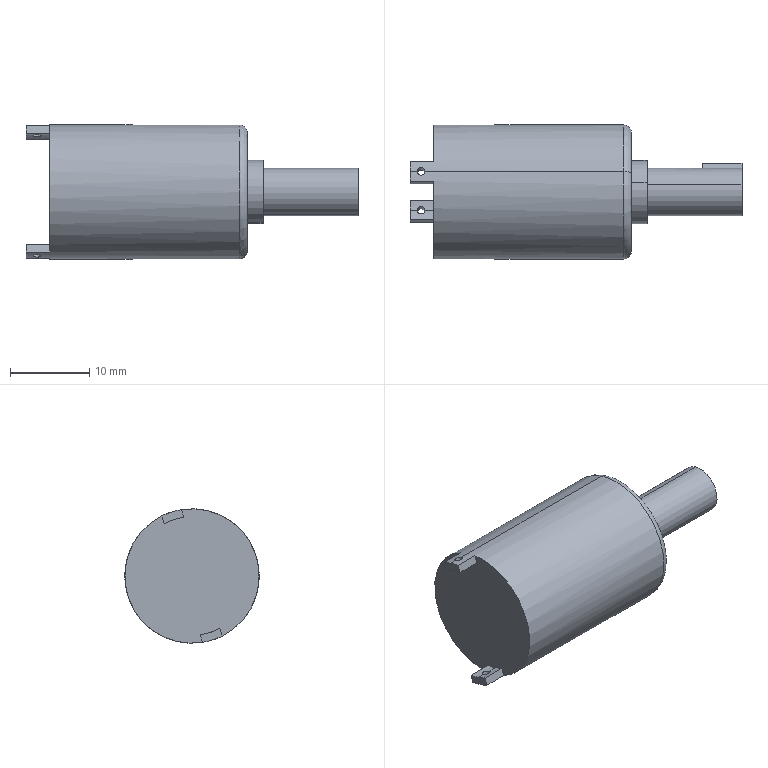Component | SolidWorks | dj-1 | 1 solid | 29 faces | box 42 x 17 x 17 mm | volume 6122 mm3 | plane 14 | cylinder 13 | torus 2 | commonest cylinder face diameters 1 x4 15 x3 6 x2 8 x2 17 x2
build123d program:
from build123d import *
from build123d.topology import SkipClean

# Parameters (mm, degrees)
SKETCH1_R           = 8.5
BOSS_EXTRUDE1_DEPTH = 25
SKETCH2_R           = 4
BOSS_EXTRUDE2_DEPTH = 2
SKETCH3_R           = 3
BOSS_EXTRUDE3_DEPTH = 12
BOSS_EXTRUDE4_START = 3
BOSS_EXTRUDE4_DEPTH = 3
SKETCH5_R           = 0.5
CUT_EXTRUDE1_DEPTH  = 31.5
FILLET1_R           = 1
SKETCH6_W           = 1.566
SKETCH6_H           = 3.572
BOSS_EXTRUDE5_DEPTH = 5


with BuildPart() as part:
    # Sketch1 → Boss-Extrude1 (new body)
    with BuildSketch(Plane.XY):
        Circle(SKETCH1_R)
    extrude(amount=BOSS_EXTRUDE1_DEPTH)

    # Sketch2 → Boss-Extrude2 (add)
    with BuildSketch(Plane.XY.offset(25)):
        Circle(SKETCH2_R)
    extrude(amount=BOSS_EXTRUDE2_DEPTH)

    # Sketch3 → Boss-Extrude3 (add)
    with BuildSketch(Plane.XY.offset(27)):
        with Locations(Location((0, 0, 0), (0, 0, 180))):
            Circle(SKETCH3_R)
    extrude(amount=BOSS_EXTRUDE3_DEPTH)

    # Sketch4 → Boss-Extrude4 (add)
    with SkipClean():  # the faces are left unmerged after this step: merging them gives an invalid solid
        with BuildSketch(Plane(origin=(0, 0, 0), x_dir=(-1, 0, 0), z_dir=(0, 0, -1)).offset(BOSS_EXTRUDE4_START)):
            with BuildLine():
                Line((-7.386, 1.303), (-8.399, 1.303))
                ThreePointArc((-8.399, 1.303), (-8.5, 0), (-8.399, -1.303))
                Line((-8.399, -1.303), (-7.386, -1.303))
                ThreePointArc((-7.386, -1.303), (-7.5, 0), (-7.386, 1.303))
            make_face()
            with BuildLine():
                Line((8.399, 1.303), (7.386, 1.303))
                ThreePointArc((7.386, 1.303), (7.5, 0), (7.386, -1.303))
                Line((7.386, -1.303), (8.399, -1.303))
                ThreePointArc((8.399, -1.303), (8.5, 0), (8.399, 1.303))
            make_face()
        extrude(amount=-BOSS_EXTRUDE4_DEPTH)

    # Sketch5 → Cut-Extrude1 (cut, symmetric)
    with SkipClean():  # the faces are left unmerged after this step: merging them gives an invalid solid
        with BuildSketch(Plane(origin=(0, 0, 0), x_dir=(0, 0, -1), z_dir=(1, 0, 0))):
            with Locations((1.599, 0)):
                Circle(SKETCH5_R)
        extrude(amount=CUT_EXTRUDE1_DEPTH, both=True, mode=Mode.SUBTRACT)

    # Fillet1
    fillet1_edges = [part.edges().sort_by_distance(p)[0] for p in [
        (-8.5, 0, 25),
    ]]
    fillet(fillet1_edges, radius=FILLET1_R)

    # Sketch6 → Boss-Extrude5 (add)
    with SkipClean():  # the faces are left unmerged after this step: merging them gives an invalid solid
        with BuildSketch(Plane.XY.offset(39)):
            with Locations((0, 1.786)):
                Rectangle(SKETCH6_W, SKETCH6_H)
        extrude(amount=-BOSS_EXTRUDE5_DEPTH)


solid = part.part

# Placed as in the assembly
solid = solid.moved(Location((24.669, 8.534, 0), (-17.868, 90, 0)))
STEP:
#1=COLOUR_RGB('',0.7922,0.8196,0.9333);
#2=FILL_AREA_STYLE_COLOUR('',#1);
#3=FILL_AREA_STYLE('',(#2));
#4=SURFACE_STYLE_FILL_AREA(#3);
#5=SURFACE_SIDE_STYLE('',(#4));
#6=SURFACE_STYLE_USAGE(.BOTH.,#5);
#7=PRESENTATION_STYLE_ASSIGNMENT((#6));
#8=CARTESIAN_POINT('',(1.916,0.4387,0.3185));
#9=VERTEX_POINT('',#8);
#10=CARTESIAN_POINT('',(1.916,0.2333,-0.3185));
#11=VERTEX_POINT('',#10);
#12=CARTESIAN_POINT('',(1.916,0.336,-0.));
#13=DIRECTION('',(-1.,0.,0.));
#14=DIRECTION('',(0.,-0.3068,-0.9518));
#15=AXIS2_PLACEMENT_3D('',#12,#13,#14);
#16=CIRCLE('',#15,0.3346);
#17=EDGE_CURVE('',#9,#11,#16,.T.);
#18=ORIENTED_EDGE('',*,*,#17,.F.);
#19=CARTESIAN_POINT('',(1.955,0.4266,0.281));
#20=VERTEX_POINT('',#19);
#21=CARTESIAN_POINT('',(1.916,0.4266,0.281));
#22=DIRECTION('',(0.,0.9518,-0.3068));
#23=DIRECTION('',(0.,0.3068,0.9518));
#24=AXIS2_PLACEMENT_3D('',#21,#22,#23);
#25=CIRCLE('',#24,0.03937);
#26=EDGE_CURVE('',#9,#20,#25,.T.);
#27=ORIENTED_EDGE('',*,*,#26,.T.);
#28=CARTESIAN_POINT('',(1.955,0.2454,-0.281));
#29=VERTEX_POINT('',#28);
#30=CARTESIAN_POINT('',(1.955,0.336,-0.));
#31=DIRECTION('',(1.,0.,0.));
#32=DIRECTION('',(0.,-0.3068,-0.9518));
#33=AXIS2_PLACEMENT_3D('',#30,#31,#32);
#34=CIRCLE('',#33,0.2953);
#35=EDGE_CURVE('',#29,#20,#34,.T.);
#36=ORIENTED_EDGE('',*,*,#35,.F.);
#37=CARTESIAN_POINT('',(1.916,0.2454,-0.281));
#38=DIRECTION('',(0.,-0.9518,0.3068));
#39=DIRECTION('',(0.,-0.3068,-0.9518));
#40=AXIS2_PLACEMENT_3D('',#37,#38,#39);
#41=CIRCLE('',#40,0.03937);
#42=EDGE_CURVE('',#11,#29,#41,.T.);
#43=ORIENTED_EDGE('',*,*,#42,.F.);
#44=EDGE_LOOP('',(#18,#27,#36,#43));
#45=FACE_OUTER_BOUND('',#44,.T.);
#46=CARTESIAN_POINT('',(1.916,0.336,-0.));
#47=DIRECTION('',(1.,0.,0.));
#48=DIRECTION('',(0.,-0.3068,-0.9518));
#49=AXIS2_PLACEMENT_3D('',#46,#47,#48);
#50=TOROIDAL_SURFACE('',#49,0.2953,0.03937);
#51=ADVANCED_FACE('',(#45),#50,.T.);
#52=CARTESIAN_POINT('',(0.928,0.4387,0.3185));
#53=VERTEX_POINT('',#52);
#54=CARTESIAN_POINT('',(0.8886,0.4387,0.3185));
#55=VERTEX_POINT('',#54);
#56=CARTESIAN_POINT('',(0.928,0.4387,0.3185));
#57=CARTESIAN_POINT('',(0.928,0.4337,0.3201));
#58=CARTESIAN_POINT('',(0.9258,0.4288,0.3215));
#59=CARTESIAN_POINT('',(0.9186,0.4218,0.3235));
#60=CARTESIAN_POINT('',(0.9134,0.4197,0.324));
#61=CARTESIAN_POINT('',(0.9031,0.4197,0.324));
#62=CARTESIAN_POINT('',(0.898,0.4218,0.3235));
#63=CARTESIAN_POINT('',(0.8907,0.4289,0.3215));
#64=CARTESIAN_POINT('',(0.8886,0.4338,0.3201));
#65=CARTESIAN_POINT('',(0.8886,0.4387,0.3185));
#66=B_SPLINE_CURVE_WITH_KNOTS('',3,(#56,#57,#58,#59,#60,#61,#62,#63,#64,#65),.UNSPECIFIED.,.F.,.F.,(4,2,2,2,4),(0.,0.0003909,0.0007818,0.001173,0.001564),.UNSPECIFIED.);
#67=EDGE_CURVE('',#53,#55,#66,.T.);
#68=ORIENTED_EDGE('',*,*,#67,.F.);
#69=CARTESIAN_POINT('',(0.928,0.4266,0.281));
#70=VERTEX_POINT('',#69);
#71=CARTESIAN_POINT('',(0.928,0.7165,1.18));
#72=DIRECTION('',(0.,-0.3068,-0.9518));
#73=VECTOR('',#72,39.37);
#74=LINE('',#71,#73);
#75=EDGE_CURVE('',#53,#70,#74,.T.);
#76=ORIENTED_EDGE('',*,*,#75,.T.);
#77=CARTESIAN_POINT('',(0.8886,0.4266,0.281));
#78=VERTEX_POINT('',#77);
#79=CARTESIAN_POINT('',(0.8886,0.4266,0.281));
#80=CARTESIAN_POINT('',(0.8886,0.4216,0.2826));
#81=CARTESIAN_POINT('',(0.8907,0.4167,0.284));
#82=CARTESIAN_POINT('',(0.898,0.4097,0.2859));
#83=CARTESIAN_POINT('',(0.9031,0.4076,0.2864));
#84=CARTESIAN_POINT('',(0.9134,0.4076,0.2864));
#85=CARTESIAN_POINT('',(0.9185,0.4097,0.286));
#86=CARTESIAN_POINT('',(0.9259,0.4168,0.284));
#87=CARTESIAN_POINT('',(0.928,0.4217,0.2826));
#88=CARTESIAN_POINT('',(0.928,0.4266,0.281));
#89=B_SPLINE_CURVE_WITH_KNOTS('',3,(#79,#80,#81,#82,#83,#84,#85,#86,#87,#88),.UNSPECIFIED.,.F.,.F.,(4,2,2,2,4),(0.,0.0003909,0.0007818,0.001173,0.001564),.UNSPECIFIED.);
#90=EDGE_CURVE('',#78,#70,#89,.T.);
#91=ORIENTED_EDGE('',*,*,#90,.F.);
#92=CARTESIAN_POINT('',(0.8886,0.7165,1.18));
#93=DIRECTION('',(0.,-0.3068,-0.9518));
#94=VECTOR('',#93,39.37);
#95=LINE('',#92,#94);
#96=EDGE_CURVE('',#55,#78,#95,.T.);
#97=ORIENTED_EDGE('',*,*,#96,.F.);
#98=EDGE_LOOP('',(#68,#76,#91,#97));
#99=FACE_OUTER_BOUND('',#98,.T.);
#100=CARTESIAN_POINT('',(0.9083,0.7165,1.18));
#101=DIRECTION('',(0.,-0.3068,-0.9518));
#102=DIRECTION('',(-1.,0.,0.));
#103=AXIS2_PLACEMENT_3D('',#100,#101,#102);
#104=CYLINDRICAL_SURFACE('',#103,0.01969);
#105=ADVANCED_FACE('',(#99),#104,.F.);
#106=CARTESIAN_POINT('',(0.928,0.2454,-0.281));
#107=VERTEX_POINT('',#106);
#108=CARTESIAN_POINT('',(0.8886,0.2454,-0.281));
#109=VERTEX_POINT('',#108);
#110=CARTESIAN_POINT('',(0.928,0.2454,-0.281));
#111=CARTESIAN_POINT('',(0.928,0.2405,-0.2795));
#112=CARTESIAN_POINT('',(0.9258,0.2357,-0.2777));
#113=CARTESIAN_POINT('',(0.9186,0.2288,-0.2752));
#114=CARTESIAN_POINT('',(0.9135,0.2269,-0.2744));
#115=CARTESIAN_POINT('',(0.9031,0.2268,-0.2744));
#116=CARTESIAN_POINT('',(0.898,0.2288,-0.2752));
#117=CARTESIAN_POINT('',(0.8907,0.2356,-0.2777));
#118=CARTESIAN_POINT('',(0.8886,0.2404,-0.2794));
#119=CARTESIAN_POINT('',(0.8886,0.2454,-0.281));
#120=B_SPLINE_CURVE_WITH_KNOTS('',3,(#110,#111,#112,#113,#114,#115,#116,#117,#118,#119),.UNSPECIFIED.,.F.,.F.,(4,2,2,2,4),(0.001564,0.001954,0.002345,0.002736,0.003127),.UNSPECIFIED.);
#121=EDGE_CURVE('',#107,#109,#120,.T.);
#122=ORIENTED_EDGE('',*,*,#121,.F.);
#123=CARTESIAN_POINT('',(0.928,0.2333,-0.3185));
#124=VERTEX_POINT('',#123);
#125=CARTESIAN_POINT('',(0.928,0.7165,1.18));
#126=DIRECTION('',(0.,-0.3068,-0.9518));
#127=VECTOR('',#126,39.37);
#128=LINE('',#125,#127);
#129=EDGE_CURVE('',#107,#124,#128,.T.);
#130=ORIENTED_EDGE('',*,*,#129,.T.);
#131=CARTESIAN_POINT('',(0.8886,0.2333,-0.3185));
#132=VERTEX_POINT('',#131);
#133=CARTESIAN_POINT('',(0.8886,0.2333,-0.3185));
#134=CARTESIAN_POINT('',(0.8886,0.2284,-0.3169));
#135=CARTESIAN_POINT('',(0.8907,0.2236,-0.3152));
#136=CARTESIAN_POINT('',(0.898,0.2167,-0.3127));
#137=CARTESIAN_POINT('',(0.9031,0.2147,-0.3119));
#138=CARTESIAN_POINT('',(0.9134,0.2147,-0.3119));
#139=CARTESIAN_POINT('',(0.9185,0.2167,-0.3127));
#140=CARTESIAN_POINT('',(0.9259,0.2236,-0.3152));
#141=CARTESIAN_POINT('',(0.928,0.2284,-0.3169));
#142=CARTESIAN_POINT('',(0.928,0.2333,-0.3185));
#143=B_SPLINE_CURVE_WITH_KNOTS('',3,(#133,#134,#135,#136,#137,#138,#139,#140,#141,#142),.UNSPECIFIED.,.F.,.F.,(4,2,2,2,4),(0.,0.0003909,0.0007818,0.001173,0.001564),.UNSPECIFIED.);
#144=EDGE_CURVE('',#132,#124,#143,.T.);
#145=ORIENTED_EDGE('',*,*,#144,.F.);
#146=CARTESIAN_POINT('',(0.8886,0.7165,1.18));
#147=DIRECTION('',(0.,-0.3068,-0.9518));
#148=VECTOR('',#147,39.37);
#149=LINE('',#146,#148);
#150=EDGE_CURVE('',#109,#132,#149,.T.);
#151=ORIENTED_EDGE('',*,*,#150,.F.);
#152=EDGE_LOOP('',(#122,#130,#145,#151));
#153=FACE_OUTER_BOUND('',#152,.T.);
#154=CARTESIAN_POINT('',(0.9083,0.7165,1.18));
#155=DIRECTION('',(0.,-0.3068,-0.9518));
#156=DIRECTION('',(-1.,0.,0.));
#157=AXIS2_PLACEMENT_3D('',#154,#155,#156);
#158=CYLINDRICAL_SURFACE('',#157,0.01969);
#159=ADVANCED_FACE('',(#153),#158,.F.);
#160=CARTESIAN_POINT('',(0.8531,0.2454,-0.281));
#161=VERTEX_POINT('',#160);
#162=CARTESIAN_POINT('',(0.8531,0.2956,-0.2925));
#163=VERTEX_POINT('',#162);
#164=CARTESIAN_POINT('',(0.8531,0.336,-0.));
#165=DIRECTION('',(1.,0.,0.));
#166=DIRECTION('',(0.,0.3068,0.9518));
#167=AXIS2_PLACEMENT_3D('',#164,#165,#166);
#168=CIRCLE('',#167,0.2953);
#169=EDGE_CURVE('',#161,#163,#168,.T.);
#170=ORIENTED_EDGE('',*,*,#169,.F.);
#171=CARTESIAN_POINT('',(0.8531,0.2454,-0.281));
#172=DIRECTION('',(1.,0.,0.));
#173=VECTOR('',#172,39.37);
#174=LINE('',#171,#173);
#175=EDGE_CURVE('',#161,#109,#174,.T.);
#176=ORIENTED_EDGE('',*,*,#175,.T.);
#177=CARTESIAN_POINT('',(0.8886,0.2454,-0.281));
#178=CARTESIAN_POINT('',(0.8886,0.2503,-0.2826));
#179=CARTESIAN_POINT('',(0.8907,0.2552,-0.284));
#180=CARTESIAN_POINT('',(0.898,0.2622,-0.2859));
#181=CARTESIAN_POINT('',(0.9031,0.2643,-0.2864));
#182=CARTESIAN_POINT('',(0.9134,0.2643,-0.2864));
#183=CARTESIAN_POINT('',(0.9185,0.2623,-0.286));
#184=CARTESIAN_POINT('',(0.9259,0.2552,-0.284));
#185=CARTESIAN_POINT('',(0.928,0.2503,-0.2826));
#186=CARTESIAN_POINT('',(0.928,0.2454,-0.281));
#187=B_SPLINE_CURVE_WITH_KNOTS('',3,(#177,#178,#179,#180,#181,#182,#183,#184,#185,#186),.UNSPECIFIED.,.F.,.F.,(4,2,2,2,4),(0.,0.0003909,0.0007818,0.001173,0.001564),.UNSPECIFIED.);
#188=EDGE_CURVE('',#109,#107,#187,.T.);
#189=ORIENTED_EDGE('',*,*,#188,.T.);
#190=CARTESIAN_POINT('',(0.9712,0.2454,-0.281));
#191=VERTEX_POINT('',#190);
#192=CARTESIAN_POINT('',(0.8531,0.2454,-0.281));
#193=DIRECTION('',(1.,0.,0.));
#194=VECTOR('',#193,39.37);
#195=LINE('',#192,#194);
#196=EDGE_CURVE('',#107,#191,#195,.T.);
#197=ORIENTED_EDGE('',*,*,#196,.T.);
#198=CARTESIAN_POINT('',(0.9712,0.2956,-0.2925));
#199=VERTEX_POINT('',#198);
#200=CARTESIAN_POINT('',(0.9712,0.336,-0.));
#201=DIRECTION('',(1.,0.,0.));
#202=DIRECTION('',(0.,0.3068,0.9518));
#203=AXIS2_PLACEMENT_3D('',#200,#201,#202);
#204=CIRCLE('',#203,0.2953);
#205=EDGE_CURVE('',#191,#199,#204,.T.);
#206=ORIENTED_EDGE('',*,*,#205,.T.);
#207=CARTESIAN_POINT('',(0.8531,0.2956,-0.2925));
#208=DIRECTION('',(1.,0.,0.));
#209=VECTOR('',#208,39.37);
#210=LINE('',#207,#209);
#211=EDGE_CURVE('',#163,#199,#210,.T.);
#212=ORIENTED_EDGE('',*,*,#211,.F.);
#213=EDGE_LOOP('',(#170,#176,#189,#197,#206,#212));
#214=FACE_OUTER_BOUND('',#213,.T.);
#215=CARTESIAN_POINT('',(0.8531,0.336,-0.));
#216=DIRECTION('',(1.,0.,0.));
#217=DIRECTION('',(0.,-0.3068,-0.9518));
#218=AXIS2_PLACEMENT_3D('',#215,#216,#217);
#219=CYLINDRICAL_SURFACE('',#218,0.2953);
#220=ADVANCED_FACE('',(#214),#219,.F.);
#221=CARTESIAN_POINT('',(2.507,0.2997,-0.1124));
#222=VERTEX_POINT('',#221);
#223=CARTESIAN_POINT('',(2.507,0.435,-0.06432));
#224=VERTEX_POINT('',#223);
#225=CARTESIAN_POINT('',(2.507,0.336,-0.));
#226=DIRECTION('',(1.,0.,0.));
#227=DIRECTION('',(0.,-0.3068,-0.9518));
#228=AXIS2_PLACEMENT_3D('',#225,#226,#227);
#229=CIRCLE('',#228,0.1181);
#230=EDGE_CURVE('',#222,#224,#229,.T.);
#231=ORIENTED_EDGE('',*,*,#230,.F.);
#232=CARTESIAN_POINT('',(2.034,0.2997,-0.1124));
#233=VERTEX_POINT('',#232);
#234=CARTESIAN_POINT('',(2.507,0.2997,-0.1124));
#235=DIRECTION('',(-1.,0.,0.));
#236=VECTOR('',#235,39.37);
#237=LINE('',#234,#236);
#238=EDGE_CURVE('',#222,#233,#237,.T.);
#239=ORIENTED_EDGE('',*,*,#238,.T.);
#240=CARTESIAN_POINT('',(2.034,0.3722,0.1124));
#241=VERTEX_POINT('',#240);
#242=CARTESIAN_POINT('',(2.034,0.336,-0.));
#243=DIRECTION('',(1.,0.,0.));
#244=DIRECTION('',(0.,-0.3068,-0.9518));
#245=AXIS2_PLACEMENT_3D('',#242,#243,#244);
#246=CIRCLE('',#245,0.1181);
#247=EDGE_CURVE('',#233,#241,#246,.T.);
#248=ORIENTED_EDGE('',*,*,#247,.T.);
#249=CARTESIAN_POINT('',(2.507,0.3722,0.1124));
#250=VERTEX_POINT('',#249);
#251=CARTESIAN_POINT('',(2.507,0.3722,0.1124));
#252=DIRECTION('',(-1.,0.,0.));
#253=VECTOR('',#252,39.37);
#254=LINE('',#251,#253);
#255=EDGE_CURVE('',#250,#241,#254,.T.);
#256=ORIENTED_EDGE('',*,*,#255,.F.);
#257=CARTESIAN_POINT('',(2.507,0.454,-0.005646));
#258=VERTEX_POINT('',#257);
#259=CARTESIAN_POINT('',(2.507,0.336,-0.));
#260=DIRECTION('',(1.,0.,0.));
#261=DIRECTION('',(0.,-0.3068,-0.9518));
#262=AXIS2_PLACEMENT_3D('',#259,#260,#261);
#263=CIRCLE('',#262,0.1181);
#264=EDGE_CURVE('',#258,#250,#263,.T.);
#265=ORIENTED_EDGE('',*,*,#264,.F.);
#266=CARTESIAN_POINT('',(2.31,0.454,-0.005646));
#267=VERTEX_POINT('',#266);
#268=CARTESIAN_POINT('',(2.507,0.454,-0.005646));
#269=DIRECTION('',(-1.,0.,0.));
#270=VECTOR('',#269,39.37);
#271=LINE('',#268,#270);
#272=EDGE_CURVE('',#258,#267,#271,.T.);
#273=ORIENTED_EDGE('',*,*,#272,.T.);
#274=CARTESIAN_POINT('',(2.31,0.435,-0.06432));
#275=VERTEX_POINT('',#274);
#276=CARTESIAN_POINT('',(2.31,0.336,-0.));
#277=DIRECTION('',(1.,0.,0.));
#278=DIRECTION('',(0.,-0.3068,-0.9518));
#279=AXIS2_PLACEMENT_3D('',#276,#277,#278);
#280=CIRCLE('',#279,0.1181);
#281=EDGE_CURVE('',#275,#267,#280,.T.);
#282=ORIENTED_EDGE('',*,*,#281,.F.);
#283=CARTESIAN_POINT('',(2.507,0.435,-0.06432));
#284=DIRECTION('',(1.,0.,0.));
#285=VECTOR('',#284,39.37);
#286=LINE('',#283,#285);
#287=EDGE_CURVE('',#275,#224,#286,.T.);
#288=ORIENTED_EDGE('',*,*,#287,.T.);
#289=EDGE_LOOP('',(#231,#239,#248,#256,#265,#273,#282,#288));
#290=FACE_OUTER_BOUND('',#289,.T.);
#291=CARTESIAN_POINT('',(2.507,0.336,-0.));
#292=DIRECTION('',(-1.,0.,0.));
#293=DIRECTION('',(0.,0.3068,0.9518));
#294=AXIS2_PLACEMENT_3D('',#291,#292,#293);
#295=CYLINDRICAL_SURFACE('',#294,0.1181);
#296=ADVANCED_FACE('',(#290),#295,.T.);
#297=CARTESIAN_POINT('',(2.034,0.2877,-0.1499));
#298=VERTEX_POINT('',#297);
#299=CARTESIAN_POINT('',(2.034,0.3843,0.1499));
#300=VERTEX_POINT('',#299);
#301=CARTESIAN_POINT('',(2.034,0.336,-0.));
#302=DIRECTION('',(1.,0.,0.));
#303=DIRECTION('',(0.,-0.3068,-0.9518));
#304=AXIS2_PLACEMENT_3D('',#301,#302,#303);
#305=CIRCLE('',#304,0.1575);
#306=EDGE_CURVE('',#298,#300,#305,.T.);
#307=ORIENTED_EDGE('',*,*,#306,.F.);
#308=CARTESIAN_POINT('',(1.955,0.2877,-0.1499));
#309=VERTEX_POINT('',#308);
#310=CARTESIAN_POINT('',(2.034,0.2877,-0.1499));
#311=DIRECTION('',(-1.,0.,0.));
#312=VECTOR('',#311,39.37);
#313=LINE('',#310,#312);
#314=EDGE_CURVE('',#298,#309,#313,.T.);
#315=ORIENTED_EDGE('',*,*,#314,.T.);
#316=CARTESIAN_POINT('',(1.955,0.3843,0.1499));
#317=VERTEX_POINT('',#316);
#318=CARTESIAN_POINT('',(1.955,0.336,-0.));
#319=DIRECTION('',(1.,0.,0.));
#320=DIRECTION('',(0.,-0.3068,-0.9518));
#321=AXIS2_PLACEMENT_3D('',#318,#319,#320);
#322=CIRCLE('',#321,0.1575);
#323=EDGE_CURVE('',#309,#317,#322,.T.);
#324=ORIENTED_EDGE('',*,*,#323,.T.);
#325=CARTESIAN_POINT('',(2.034,0.3843,0.1499));
#326=DIRECTION('',(-1.,0.,0.));
#327=VECTOR('',#326,39.37);
#328=LINE('',#325,#327);
#329=EDGE_CURVE('',#300,#317,#328,.T.);
#330=ORIENTED_EDGE('',*,*,#329,.F.);
#331=EDGE_LOOP('',(#307,#315,#324,#330));
#332=FACE_OUTER_BOUND('',#331,.T.);
#333=CARTESIAN_POINT('',(2.034,0.336,-0.));
#334=DIRECTION('',(-1.,0.,0.));
#335=DIRECTION('',(0.,0.3068,0.9518));
#336=AXIS2_PLACEMENT_3D('',#333,#334,#335);
#337=CYLINDRICAL_SURFACE('',#336,0.1575);
#338=ADVANCED_FACE('',(#332),#337,.T.);
#339=ORIENTED_EDGE('',*,*,#17,.T.);
#340=CARTESIAN_POINT('',(1.955,0.2333,-0.3185));
#341=DIRECTION('',(-1.,0.,0.));
#342=VECTOR('',#341,39.37);
#343=LINE('',#340,#342);
#344=EDGE_CURVE('',#11,#124,#343,.T.);
#345=ORIENTED_EDGE('',*,*,#344,.T.);
#346=CARTESIAN_POINT('',(0.928,0.2333,-0.3185));
#347=CARTESIAN_POINT('',(0.928,0.2382,-0.3201));
#348=CARTESIAN_POINT('',(0.9258,0.2431,-0.3215));
#349=CARTESIAN_POINT('',(0.9186,0.2501,-0.3235));
#350=CARTESIAN_POINT('',(0.9135,0.2522,-0.324));
#351=CARTESIAN_POINT('',(0.9031,0.2522,-0.324));
#352=CARTESIAN_POINT('',(0.898,0.2502,-0.3235));
#353=CARTESIAN_POINT('',(0.8907,0.2431,-0.3215));
#354=CARTESIAN_POINT('',(0.8886,0.2383,-0.3201));
#355=CARTESIAN_POINT('',(0.8886,0.2333,-0.3185));
#356=B_SPLINE_CURVE_WITH_KNOTS('',3,(#346,#347,#348,#349,#350,#351,#352,#353,#354,#355),.UNSPECIFIED.,.F.,.F.,(4,2,2,2,4),(0.001564,0.001954,0.002345,0.002736,0.003127),.UNSPECIFIED.);
#357=EDGE_CURVE('',#124,#132,#356,.T.);
#358=ORIENTED_EDGE('',*,*,#357,.T.);
#359=CARTESIAN_POINT('',(0.8531,0.2333,-0.3185));
#360=VERTEX_POINT('',#359);
#361=CARTESIAN_POINT('',(1.955,0.2333,-0.3185));
#362=DIRECTION('',(-1.,0.,0.));
#363=VECTOR('',#362,39.37);
#364=LINE('',#361,#363);
#365=EDGE_CURVE('',#132,#360,#364,.T.);
#366=ORIENTED_EDGE('',*,*,#365,.T.);
#367=CARTESIAN_POINT('',(0.8531,0.2834,-0.3305));
#368=VERTEX_POINT('',#367);
#369=CARTESIAN_POINT('',(0.8531,0.336,-0.));
#370=DIRECTION('',(-1.,0.,0.));
#371=DIRECTION('',(0.,0.3068,0.9518));
#372=AXIS2_PLACEMENT_3D('',#369,#370,#371);
#373=CIRCLE('',#372,0.3346);
#374=EDGE_CURVE('',#368,#360,#373,.T.);
#375=ORIENTED_EDGE('',*,*,#374,.F.);
#376=CARTESIAN_POINT('',(0.9712,0.2834,-0.3305));
#377=VERTEX_POINT('',#376);
#378=CARTESIAN_POINT('',(0.8531,0.2834,-0.3305));
#379=DIRECTION('',(1.,0.,0.));
#380=VECTOR('',#379,39.37);
#381=LINE('',#378,#380);
#382=EDGE_CURVE('',#368,#377,#381,.T.);
#383=ORIENTED_EDGE('',*,*,#382,.T.);
#384=CARTESIAN_POINT('',(0.9712,0.4863,0.299));
#385=VERTEX_POINT('',#384);
#386=CARTESIAN_POINT('',(0.9712,0.336,-0.));
#387=DIRECTION('',(1.,0.,0.));
#388=DIRECTION('',(0.,-0.3068,-0.9518));
#389=AXIS2_PLACEMENT_3D('',#386,#387,#388);
#390=CIRCLE('',#389,0.3346);
#391=EDGE_CURVE('',#377,#385,#390,.T.);
#392=ORIENTED_EDGE('',*,*,#391,.T.);
#393=CARTESIAN_POINT('',(0.8531,0.4863,0.299));
#394=VERTEX_POINT('',#393);
#395=CARTESIAN_POINT('',(0.8531,0.4863,0.299));
#396=DIRECTION('',(1.,0.,0.));
#397=VECTOR('',#396,39.37);
#398=LINE('',#395,#397);
#399=EDGE_CURVE('',#394,#385,#398,.T.);
#400=ORIENTED_EDGE('',*,*,#399,.F.);
#401=CARTESIAN_POINT('',(0.8531,0.4387,0.3185));
#402=VERTEX_POINT('',#401);
#403=CARTESIAN_POINT('',(0.8531,0.336,-0.));
#404=DIRECTION('',(-1.,0.,0.));
#405=DIRECTION('',(0.,0.3068,0.9518));
#406=AXIS2_PLACEMENT_3D('',#403,#404,#405);
#407=CIRCLE('',#406,0.3346);
#408=EDGE_CURVE('',#402,#394,#407,.T.);
#409=ORIENTED_EDGE('',*,*,#408,.F.);
#410=CARTESIAN_POINT('',(1.955,0.4387,0.3185));
#411=DIRECTION('',(-1.,0.,0.));
#412=VECTOR('',#411,39.37);
#413=LINE('',#410,#412);
#414=EDGE_CURVE('',#55,#402,#413,.T.);
#415=ORIENTED_EDGE('',*,*,#414,.F.);
#416=CARTESIAN_POINT('',(0.8886,0.4387,0.3185));
#417=CARTESIAN_POINT('',(0.8886,0.4436,0.3169));
#418=CARTESIAN_POINT('',(0.8907,0.4484,0.3152));
#419=CARTESIAN_POINT('',(0.898,0.4552,0.3127));
#420=CARTESIAN_POINT('',(0.9031,0.4572,0.3119));
#421=CARTESIAN_POINT('',(0.9135,0.4572,0.3119));
#422=CARTESIAN_POINT('',(0.9185,0.4552,0.3127));
#423=CARTESIAN_POINT('',(0.9258,0.4484,0.3152));
#424=CARTESIAN_POINT('',(0.928,0.4436,0.3169));
#425=CARTESIAN_POINT('',(0.928,0.4387,0.3185));
#426=B_SPLINE_CURVE_WITH_KNOTS('',3,(#416,#417,#418,#419,#420,#421,#422,#423,#424,#425),.UNSPECIFIED.,.F.,.F.,(4,2,2,2,4),(0.001564,0.001954,0.002345,0.002736,0.003127),.UNSPECIFIED.);
#427=EDGE_CURVE('',#55,#53,#426,.T.);
#428=ORIENTED_EDGE('',*,*,#427,.T.);
#429=CARTESIAN_POINT('',(1.955,0.4387,0.3185));
#430=DIRECTION('',(-1.,0.,0.));
#431=VECTOR('',#430,39.37);
#432=LINE('',#429,#431);
#433=EDGE_CURVE('',#9,#53,#432,.T.);
#434=ORIENTED_EDGE('',*,*,#433,.F.);
#435=EDGE_LOOP('',(#339,#345,#358,#366,#375,#383,#392,#400,#409,#415,#428,#434));
#436=FACE_OUTER_BOUND('',#435,.T.);
#437=CARTESIAN_POINT('',(1.955,0.336,-0.));
#438=DIRECTION('',(-1.,0.,0.));
#439=DIRECTION('',(0.,0.3068,0.9518));
#440=AXIS2_PLACEMENT_3D('',#437,#438,#439);
#441=CYLINDRICAL_SURFACE('',#440,0.3346);
#442=ADVANCED_FACE('',(#436),#441,.T.);
#443=CARTESIAN_POINT('',(0.9712,0.1857,-0.299));
#444=VERTEX_POINT('',#443);
#445=CARTESIAN_POINT('',(0.9712,0.1979,-0.261));
#446=VERTEX_POINT('',#445);
#447=CARTESIAN_POINT('',(0.9712,0.1979,-0.261));
#448=DIRECTION('',(0.,0.3068,0.9518));
#449=VECTOR('',#448,39.37);
#450=LINE('',#447,#449);
#451=EDGE_CURVE('',#444,#446,#450,.T.);
#452=ORIENTED_EDGE('',*,*,#451,.F.);
#453=CARTESIAN_POINT('',(0.9712,0.3886,0.3305));
#454=VERTEX_POINT('',#453);
#455=CARTESIAN_POINT('',(0.9712,0.336,-0.));
#456=DIRECTION('',(1.,0.,0.));
#457=DIRECTION('',(0.,-0.3068,-0.9518));
#458=AXIS2_PLACEMENT_3D('',#455,#456,#457);
#459=CIRCLE('',#458,0.3346);
#460=EDGE_CURVE('',#454,#444,#459,.T.);
#461=ORIENTED_EDGE('',*,*,#460,.F.);
#462=CARTESIAN_POINT('',(0.9712,0.3764,0.2925));
#463=VERTEX_POINT('',#462);
#464=CARTESIAN_POINT('',(0.9712,0.3886,0.3305));
#465=DIRECTION('',(0.,0.3068,0.9518));
#466=VECTOR('',#465,39.37);
#467=LINE('',#464,#466);
#468=EDGE_CURVE('',#463,#454,#467,.T.);
#469=ORIENTED_EDGE('',*,*,#468,.F.);
#470=CARTESIAN_POINT('',(0.9712,0.474,0.261));
#471=VERTEX_POINT('',#470);
#472=CARTESIAN_POINT('',(0.9712,0.336,-0.));
#473=DIRECTION('',(1.,0.,0.));
#474=DIRECTION('',(0.,0.3068,0.9518));
#475=AXIS2_PLACEMENT_3D('',#472,#473,#474);
#476=CIRCLE('',#475,0.2953);
#477=EDGE_CURVE('',#471,#463,#476,.T.);
#478=ORIENTED_EDGE('',*,*,#477,.F.);
#479=CARTESIAN_POINT('',(0.9712,0.4863,0.299));
#480=DIRECTION('',(0.,-0.3068,-0.9518));
#481=VECTOR('',#480,39.37);
#482=LINE('',#479,#481);
#483=EDGE_CURVE('',#385,#471,#482,.T.);
#484=ORIENTED_EDGE('',*,*,#483,.F.);
#485=ORIENTED_EDGE('',*,*,#391,.F.);
#486=CARTESIAN_POINT('',(0.9712,0.2956,-0.2925));
#487=DIRECTION('',(0.,-0.3068,-0.9518));
#488=VECTOR('',#487,39.37);
#489=LINE('',#486,#488);
#490=EDGE_CURVE('',#199,#377,#489,.T.);
#491=ORIENTED_EDGE('',*,*,#490,.F.);
#492=ORIENTED_EDGE('',*,*,#205,.F.);
#493=CARTESIAN_POINT('',(0.9712,0.336,-0.));
#494=DIRECTION('',(1.,0.,0.));
#495=DIRECTION('',(0.,0.3068,0.9518));
#496=AXIS2_PLACEMENT_3D('',#493,#494,#495);
#497=CIRCLE('',#496,0.2953);
#498=EDGE_CURVE('',#446,#191,#497,.T.);
#499=ORIENTED_EDGE('',*,*,#498,.F.);
#500=EDGE_LOOP('',(#452,#461,#469,#478,#484,#485,#491,#492,#499));
#501=FACE_OUTER_BOUND('',#500,.T.);
#502=CARTESIAN_POINT('',(0.9712,0.336,-0.));
#503=DIRECTION('',(1.,0.,0.));
#504=DIRECTION('',(0.,-0.3068,-0.9518));
#505=AXIS2_PLACEMENT_3D('',#502,#503,#504);
#506=PLANE('',#505);
#507=ADVANCED_FACE('',(#501),#506,.F.);
#508=CARTESIAN_POINT('',(2.034,0.336,-0.));
#509=DIRECTION('',(1.,0.,0.));
#510=DIRECTION('',(0.,-0.3068,-0.9518));
#511=AXIS2_PLACEMENT_3D('',#508,#509,#510);
#512=CIRCLE('',#511,0.1575);
#513=EDGE_CURVE('',#300,#298,#512,.T.);
#514=ORIENTED_EDGE('',*,*,#513,.T.);
#515=ORIENTED_EDGE('',*,*,#306,.T.);
#516=EDGE_LOOP('',(#514,#515));
#517=FACE_OUTER_BOUND('',#516,.T.);
#518=CARTESIAN_POINT('',(2.034,0.336,-0.));
#519=DIRECTION('',(1.,0.,0.));
#520=DIRECTION('',(0.,-0.3068,-0.9518));
#521=AXIS2_PLACEMENT_3D('',#518,#519,#520);
#522=CIRCLE('',#521,0.1181);
#523=EDGE_CURVE('',#241,#233,#522,.T.);
#524=ORIENTED_EDGE('',*,*,#523,.F.);
#525=ORIENTED_EDGE('',*,*,#247,.F.);
#526=EDGE_LOOP('',(#524,#525));
#527=FACE_BOUND('',#526,.T.);
#528=CARTESIAN_POINT('',(2.034,0.336,-0.));
#529=DIRECTION('',(1.,0.,0.));
#530=DIRECTION('',(0.,-0.3068,-0.9518));
#531=AXIS2_PLACEMENT_3D('',#528,#529,#530);
#532=PLANE('',#531);
#533=ADVANCED_FACE('',(#517,#527),#532,.T.);
#534=ORIENTED_EDGE('',*,*,#35,.T.);
#535=CARTESIAN_POINT('',(1.955,0.336,-0.));
#536=DIRECTION('',(1.,0.,0.));
#537=DIRECTION('',(0.,-0.3068,-0.9518));
#538=AXIS2_PLACEMENT_3D('',#535,#536,#537);
#539=CIRCLE('',#538,0.2953);
#540=EDGE_CURVE('',#20,#29,#539,.T.);
#541=ORIENTED_EDGE('',*,*,#540,.T.);
#542=EDGE_LOOP('',(#534,#541));
#543=FACE_OUTER_BOUND('',#542,.T.);
#544=CARTESIAN_POINT('',(1.955,0.336,-0.));
#545=DIRECTION('',(1.,0.,0.));
#546=DIRECTION('',(0.,-0.3068,-0.9518));
#547=AXIS2_PLACEMENT_3D('',#544,#545,#546);
#548=CIRCLE('',#547,0.1575);
#549=EDGE_CURVE('',#317,#309,#548,.T.);
#550=ORIENTED_EDGE('',*,*,#549,.F.);
#551=ORIENTED_EDGE('',*,*,#323,.F.);
#552=EDGE_LOOP('',(#550,#551));
#553=FACE_BOUND('',#552,.T.);
#554=CARTESIAN_POINT('',(1.955,0.336,-0.));
#555=DIRECTION('',(1.,0.,0.));
#556=DIRECTION('',(0.,-0.3068,-0.9518));
#557=AXIS2_PLACEMENT_3D('',#554,#555,#556);
#558=PLANE('',#557);
#559=ADVANCED_FACE('',(#543,#553),#558,.T.);
#560=ORIENTED_EDGE('',*,*,#344,.F.);
#561=CARTESIAN_POINT('',(1.916,0.336,-0.));
#562=DIRECTION('',(-1.,0.,0.));
#563=DIRECTION('',(0.,-0.3068,-0.9518));
#564=AXIS2_PLACEMENT_3D('',#561,#562,#563);
#565=CIRCLE('',#564,0.3346);
#566=EDGE_CURVE('',#11,#9,#565,.T.);
#567=ORIENTED_EDGE('',*,*,#566,.T.);
#568=ORIENTED_EDGE('',*,*,#433,.T.);
#569=ORIENTED_EDGE('',*,*,#67,.T.);
#570=ORIENTED_EDGE('',*,*,#414,.T.);
#571=CARTESIAN_POINT('',(0.8531,0.3886,0.3305));
#572=VERTEX_POINT('',#571);
#573=CARTESIAN_POINT('',(0.8531,0.336,-0.));
#574=DIRECTION('',(-1.,0.,0.));
#575=DIRECTION('',(0.,0.3068,0.9518));
#576=AXIS2_PLACEMENT_3D('',#573,#574,#575);
#577=CIRCLE('',#576,0.3346);
#578=EDGE_CURVE('',#572,#402,#577,.T.);
#579=ORIENTED_EDGE('',*,*,#578,.F.);
#580=CARTESIAN_POINT('',(0.8531,0.3886,0.3305));
#581=DIRECTION('',(1.,0.,0.));
#582=VECTOR('',#581,39.37);
#583=LINE('',#580,#582);
#584=EDGE_CURVE('',#572,#454,#583,.T.);
#585=ORIENTED_EDGE('',*,*,#584,.T.);
#586=ORIENTED_EDGE('',*,*,#460,.T.);
#587=CARTESIAN_POINT('',(0.8531,0.1857,-0.299));
#588=VERTEX_POINT('',#587);
#589=CARTESIAN_POINT('',(0.8531,0.1857,-0.299));
#590=DIRECTION('',(1.,0.,0.));
#591=VECTOR('',#590,39.37);
#592=LINE('',#589,#591);
#593=EDGE_CURVE('',#588,#444,#592,.T.);
#594=ORIENTED_EDGE('',*,*,#593,.F.);
#595=CARTESIAN_POINT('',(0.8531,0.336,-0.));
#596=DIRECTION('',(-1.,0.,0.));
#597=DIRECTION('',(0.,0.3068,0.9518));
#598=AXIS2_PLACEMENT_3D('',#595,#596,#597);
#599=CIRCLE('',#598,0.3346);
#600=EDGE_CURVE('',#360,#588,#599,.T.);
#601=ORIENTED_EDGE('',*,*,#600,.F.);
#602=ORIENTED_EDGE('',*,*,#365,.F.);
#603=ORIENTED_EDGE('',*,*,#144,.T.);
#604=EDGE_LOOP('',(#560,#567,#568,#569,#570,#579,#585,#586,#594,#601,#602,#603));
#605=FACE_OUTER_BOUND('',#604,.T.);
#606=CARTESIAN_POINT('',(1.955,0.336,-0.));
#607=DIRECTION('',(-1.,0.,0.));
#608=DIRECTION('',(0.,0.3068,0.9518));
#609=AXIS2_PLACEMENT_3D('',#606,#607,#608);
#610=CYLINDRICAL_SURFACE('',#609,0.3346);
#611=ADVANCED_FACE('',(#605),#610,.T.);
#612=ORIENTED_EDGE('',*,*,#314,.F.);
#613=ORIENTED_EDGE('',*,*,#513,.F.);
#614=ORIENTED_EDGE('',*,*,#329,.T.);
#615=ORIENTED_EDGE('',*,*,#549,.T.);
#616=EDGE_LOOP('',(#612,#613,#614,#615));
#617=FACE_OUTER_BOUND('',#616,.T.);
#618=CARTESIAN_POINT('',(2.034,0.336,-0.));
#619=DIRECTION('',(-1.,0.,0.));
#620=DIRECTION('',(0.,0.3068,0.9518));
#621=AXIS2_PLACEMENT_3D('',#618,#619,#620);
#622=CYLINDRICAL_SURFACE('',#621,0.1575);
#623=ADVANCED_FACE('',(#617),#622,.T.);
#624=ORIENTED_EDGE('',*,*,#238,.F.);
#625=CARTESIAN_POINT('',(2.507,0.336,-0.));
#626=DIRECTION('',(1.,0.,0.));
#627=DIRECTION('',(0.,-0.3068,-0.9518));
#628=AXIS2_PLACEMENT_3D('',#625,#626,#627);
#629=CIRCLE('',#628,0.1181);
#630=EDGE_CURVE('',#250,#222,#629,.T.);
#631=ORIENTED_EDGE('',*,*,#630,.F.);
#632=ORIENTED_EDGE('',*,*,#255,.T.);
#633=ORIENTED_EDGE('',*,*,#523,.T.);
#634=EDGE_LOOP('',(#624,#631,#632,#633));
#635=FACE_OUTER_BOUND('',#634,.T.);
#636=CARTESIAN_POINT('',(2.507,0.336,-0.));
#637=DIRECTION('',(-1.,0.,0.));
#638=DIRECTION('',(0.,0.3068,0.9518));
#639=AXIS2_PLACEMENT_3D('',#636,#637,#638);
#640=CYLINDRICAL_SURFACE('',#639,0.1181);
#641=ADVANCED_FACE('',(#635),#640,.T.);
#642=ORIENTED_EDGE('',*,*,#264,.T.);
#643=ORIENTED_EDGE('',*,*,#630,.T.);
#644=ORIENTED_EDGE('',*,*,#230,.T.);
#645=CARTESIAN_POINT('',(2.507,0.4604,-0.07249));
#646=VERTEX_POINT('',#645);
#647=CARTESIAN_POINT('',(2.507,0.3265,-0.02934));
#648=DIRECTION('',(0.,0.9518,-0.3068));
#649=VECTOR('',#648,39.37);
#650=LINE('',#647,#649);
#651=EDGE_CURVE('',#224,#646,#650,.T.);
#652=ORIENTED_EDGE('',*,*,#651,.T.);
#653=CARTESIAN_POINT('',(2.507,0.4793,-0.01382));
#654=VERTEX_POINT('',#653);
#655=CARTESIAN_POINT('',(2.507,0.4604,-0.07249));
#656=DIRECTION('',(0.,0.3068,0.9518));
#657=VECTOR('',#656,39.37);
#658=LINE('',#655,#657);
#659=EDGE_CURVE('',#646,#654,#658,.T.);
#660=ORIENTED_EDGE('',*,*,#659,.T.);
#661=CARTESIAN_POINT('',(2.507,0.3454,0.02934));
#662=DIRECTION('',(0.,-0.9518,0.3068));
#663=VECTOR('',#662,39.37);
#664=LINE('',#661,#663);
#665=EDGE_CURVE('',#654,#258,#664,.T.);
#666=ORIENTED_EDGE('',*,*,#665,.T.);
#667=EDGE_LOOP('',(#642,#643,#644,#652,#660,#666));
#668=FACE_OUTER_BOUND('',#667,.T.);
#669=CARTESIAN_POINT('',(2.507,0.336,-0.));
#670=DIRECTION('',(1.,0.,0.));
#671=DIRECTION('',(0.,-0.3068,-0.9518));
#672=AXIS2_PLACEMENT_3D('',#669,#670,#671);
#673=PLANE('',#672);
#674=ADVANCED_FACE('',(#668),#673,.T.);
#675=ORIENTED_EDGE('',*,*,#90,.T.);
#676=CARTESIAN_POINT('',(0.928,0.4266,0.281));
#677=CARTESIAN_POINT('',(0.928,0.4315,0.2795));
#678=CARTESIAN_POINT('',(0.9258,0.4363,0.2777));
#679=CARTESIAN_POINT('',(0.9186,0.4431,0.2752));
#680=CARTESIAN_POINT('',(0.9135,0.4451,0.2744));
#681=CARTESIAN_POINT('',(0.9031,0.4451,0.2744));
#682=CARTESIAN_POINT('',(0.898,0.4431,0.2752));
#683=CARTESIAN_POINT('',(0.8907,0.4363,0.2777));
#684=CARTESIAN_POINT('',(0.8886,0.4315,0.2794));
#685=CARTESIAN_POINT('',(0.8886,0.4266,0.281));
#686=B_SPLINE_CURVE_WITH_KNOTS('',3,(#676,#677,#678,#679,#680,#681,#682,#683,#684,#685),.UNSPECIFIED.,.F.,.F.,(4,2,2,2,4),(0.001564,0.001954,0.002345,0.002736,0.003127),.UNSPECIFIED.);
#687=EDGE_CURVE('',#70,#78,#686,.T.);
#688=ORIENTED_EDGE('',*,*,#687,.T.);
#689=EDGE_LOOP('',(#675,#688));
#690=FACE_BOUND('',#689,.T.);
#691=ORIENTED_EDGE('',*,*,#477,.T.);
#692=CARTESIAN_POINT('',(0.8531,0.3764,0.2925));
#693=VERTEX_POINT('',#692);
#694=CARTESIAN_POINT('',(0.8531,0.3764,0.2925));
#695=DIRECTION('',(1.,0.,0.));
#696=VECTOR('',#695,39.37);
#697=LINE('',#694,#696);
#698=EDGE_CURVE('',#693,#463,#697,.T.);
#699=ORIENTED_EDGE('',*,*,#698,.F.);
#700=CARTESIAN_POINT('',(0.8531,0.474,0.261));
#701=VERTEX_POINT('',#700);
#702=CARTESIAN_POINT('',(0.8531,0.336,-0.));
#703=DIRECTION('',(1.,0.,0.));
#704=DIRECTION('',(0.,0.3068,0.9518));
#705=AXIS2_PLACEMENT_3D('',#702,#703,#704);
#706=CIRCLE('',#705,0.2953);
#707=EDGE_CURVE('',#701,#693,#706,.T.);
#708=ORIENTED_EDGE('',*,*,#707,.F.);
#709=CARTESIAN_POINT('',(0.8531,0.474,0.261));
#710=DIRECTION('',(1.,0.,0.));
#711=VECTOR('',#710,39.37);
#712=LINE('',#709,#711);
#713=EDGE_CURVE('',#701,#471,#712,.T.);
#714=ORIENTED_EDGE('',*,*,#713,.T.);
#715=EDGE_LOOP('',(#691,#699,#708,#714));
#716=FACE_OUTER_BOUND('',#715,.T.);
#717=CARTESIAN_POINT('',(0.8531,0.336,-0.));
#718=DIRECTION('',(1.,0.,0.));
#719=DIRECTION('',(0.,-0.3068,-0.9518));
#720=AXIS2_PLACEMENT_3D('',#717,#718,#719);
#721=CYLINDRICAL_SURFACE('',#720,0.2953);
#722=ADVANCED_FACE('',(#690,#716),#721,.F.);
#723=ORIENTED_EDGE('',*,*,#468,.T.);
#724=ORIENTED_EDGE('',*,*,#584,.F.);
#725=CARTESIAN_POINT('',(0.8531,0.3886,0.3305));
#726=DIRECTION('',(0.,0.3068,0.9518));
#727=VECTOR('',#726,39.37);
#728=LINE('',#725,#727);
#729=EDGE_CURVE('',#693,#572,#728,.T.);
#730=ORIENTED_EDGE('',*,*,#729,.F.);
#731=ORIENTED_EDGE('',*,*,#698,.T.);
#732=EDGE_LOOP('',(#723,#724,#730,#731));
#733=FACE_OUTER_BOUND('',#732,.T.);
#734=CARTESIAN_POINT('',(0.8531,0.3886,0.3305));
#735=DIRECTION('',(0.,0.9518,-0.3068));
#736=DIRECTION('',(1.,0.,0.));
#737=AXIS2_PLACEMENT_3D('',#734,#735,#736);
#738=PLANE('',#737);
#739=ADVANCED_FACE('',(#733),#738,.F.);
#740=ORIENTED_EDGE('',*,*,#483,.T.);
#741=ORIENTED_EDGE('',*,*,#713,.F.);
#742=CARTESIAN_POINT('',(0.8531,0.4863,0.299));
#743=DIRECTION('',(0.,-0.3068,-0.9518));
#744=VECTOR('',#743,39.37);
#745=LINE('',#742,#744);
#746=EDGE_CURVE('',#394,#701,#745,.T.);
#747=ORIENTED_EDGE('',*,*,#746,.F.);
#748=ORIENTED_EDGE('',*,*,#399,.T.);
#749=EDGE_LOOP('',(#740,#741,#747,#748));
#750=FACE_OUTER_BOUND('',#749,.T.);
#751=CARTESIAN_POINT('',(0.8531,0.4863,0.299));
#752=DIRECTION('',(0.,-0.9518,0.3068));
#753=DIRECTION('',(-1.,0.,0.));
#754=AXIS2_PLACEMENT_3D('',#751,#752,#753);
#755=PLANE('',#754);
#756=ADVANCED_FACE('',(#750),#755,.F.);
#757=ORIENTED_EDGE('',*,*,#707,.T.);
#758=ORIENTED_EDGE('',*,*,#729,.T.);
#759=ORIENTED_EDGE('',*,*,#578,.T.);
#760=ORIENTED_EDGE('',*,*,#408,.T.);
#761=ORIENTED_EDGE('',*,*,#746,.T.);
#762=EDGE_LOOP('',(#757,#758,#759,#760,#761));
#763=FACE_OUTER_BOUND('',#762,.T.);
#764=CARTESIAN_POINT('',(0.8531,0.336,-0.));
#765=DIRECTION('',(-1.,0.,0.));
#766=DIRECTION('',(0.,0.3068,0.9518));
#767=AXIS2_PLACEMENT_3D('',#764,#765,#766);
#768=PLANE('',#767);
#769=ADVANCED_FACE('',(#763),#768,.T.);
#770=ORIENTED_EDGE('',*,*,#451,.T.);
#771=CARTESIAN_POINT('',(0.8531,0.1979,-0.261));
#772=VERTEX_POINT('',#771);
#773=CARTESIAN_POINT('',(0.8531,0.1979,-0.261));
#774=DIRECTION('',(1.,0.,0.));
#775=VECTOR('',#774,39.37);
#776=LINE('',#773,#775);
#777=EDGE_CURVE('',#772,#446,#776,.T.);
#778=ORIENTED_EDGE('',*,*,#777,.F.);
#779=CARTESIAN_POINT('',(0.8531,0.1979,-0.261));
#780=DIRECTION('',(0.,0.3068,0.9518));
#781=VECTOR('',#780,39.37);
#782=LINE('',#779,#781);
#783=EDGE_CURVE('',#588,#772,#782,.T.);
#784=ORIENTED_EDGE('',*,*,#783,.F.);
#785=ORIENTED_EDGE('',*,*,#593,.T.);
#786=EDGE_LOOP('',(#770,#778,#784,#785));
#787=FACE_OUTER_BOUND('',#786,.T.);
#788=CARTESIAN_POINT('',(0.8531,0.1979,-0.261));
#789=DIRECTION('',(0.,0.9518,-0.3068));
#790=DIRECTION('',(1.,0.,0.));
#791=AXIS2_PLACEMENT_3D('',#788,#789,#790);
#792=PLANE('',#791);
#793=ADVANCED_FACE('',(#787),#792,.F.);
#794=ORIENTED_EDGE('',*,*,#175,.F.);
#795=CARTESIAN_POINT('',(0.8531,0.336,-0.));
#796=DIRECTION('',(1.,0.,0.));
#797=DIRECTION('',(0.,0.3068,0.9518));
#798=AXIS2_PLACEMENT_3D('',#795,#796,#797);
#799=CIRCLE('',#798,0.2953);
#800=EDGE_CURVE('',#772,#161,#799,.T.);
#801=ORIENTED_EDGE('',*,*,#800,.F.);
#802=ORIENTED_EDGE('',*,*,#777,.T.);
#803=ORIENTED_EDGE('',*,*,#498,.T.);
#804=ORIENTED_EDGE('',*,*,#196,.F.);
#805=ORIENTED_EDGE('',*,*,#121,.T.);
#806=EDGE_LOOP('',(#794,#801,#802,#803,#804,#805));
#807=FACE_OUTER_BOUND('',#806,.T.);
#808=CARTESIAN_POINT('',(0.8531,0.336,-0.));
#809=DIRECTION('',(1.,0.,0.));
#810=DIRECTION('',(0.,-0.3068,-0.9518));
#811=AXIS2_PLACEMENT_3D('',#808,#809,#810);
#812=CYLINDRICAL_SURFACE('',#811,0.2953);
#813=ADVANCED_FACE('',(#807),#812,.F.);
#814=ORIENTED_EDGE('',*,*,#490,.T.);
#815=ORIENTED_EDGE('',*,*,#382,.F.);
#816=CARTESIAN_POINT('',(0.8531,0.2956,-0.2925));
#817=DIRECTION('',(0.,-0.3068,-0.9518));
#818=VECTOR('',#817,39.37);
#819=LINE('',#816,#818);
#820=EDGE_CURVE('',#163,#368,#819,.T.);
#821=ORIENTED_EDGE('',*,*,#820,.F.);
#822=ORIENTED_EDGE('',*,*,#211,.T.);
#823=EDGE_LOOP('',(#814,#815,#821,#822));
#824=FACE_OUTER_BOUND('',#823,.T.);
#825=CARTESIAN_POINT('',(0.8531,0.2956,-0.2925));
#826=DIRECTION('',(0.,-0.9518,0.3068));
#827=DIRECTION('',(-1.,0.,0.));
#828=AXIS2_PLACEMENT_3D('',#825,#826,#827);
#829=PLANE('',#828);
#830=ADVANCED_FACE('',(#824),#829,.F.);
#831=ORIENTED_EDGE('',*,*,#374,.T.);
#832=ORIENTED_EDGE('',*,*,#600,.T.);
#833=ORIENTED_EDGE('',*,*,#783,.T.);
#834=ORIENTED_EDGE('',*,*,#800,.T.);
#835=ORIENTED_EDGE('',*,*,#169,.T.);
#836=ORIENTED_EDGE('',*,*,#820,.T.);
#837=EDGE_LOOP('',(#831,#832,#833,#834,#835,#836));
#838=FACE_OUTER_BOUND('',#837,.T.);
#839=CARTESIAN_POINT('',(0.8531,0.336,-0.));
#840=DIRECTION('',(-1.,0.,0.));
#841=DIRECTION('',(0.,0.3068,0.9518));
#842=AXIS2_PLACEMENT_3D('',#839,#840,#841);
#843=PLANE('',#842);
#844=ADVANCED_FACE('',(#838),#843,.T.);
#845=ORIENTED_EDGE('',*,*,#129,.F.);
#846=ORIENTED_EDGE('',*,*,#188,.F.);
#847=ORIENTED_EDGE('',*,*,#150,.T.);
#848=ORIENTED_EDGE('',*,*,#357,.F.);
#849=EDGE_LOOP('',(#845,#846,#847,#848));
#850=FACE_OUTER_BOUND('',#849,.T.);
#851=CARTESIAN_POINT('',(0.9083,0.7165,1.18));
#852=DIRECTION('',(0.,-0.3068,-0.9518));
#853=DIRECTION('',(-1.,0.,0.));
#854=AXIS2_PLACEMENT_3D('',#851,#852,#853);
#855=CYLINDRICAL_SURFACE('',#854,0.01969);
#856=ADVANCED_FACE('',(#850),#855,.F.);
#857=ORIENTED_EDGE('',*,*,#75,.F.);
#858=ORIENTED_EDGE('',*,*,#427,.F.);
#859=ORIENTED_EDGE('',*,*,#96,.T.);
#860=ORIENTED_EDGE('',*,*,#687,.F.);
#861=EDGE_LOOP('',(#857,#858,#859,#860));
#862=FACE_OUTER_BOUND('',#861,.T.);
#863=CARTESIAN_POINT('',(0.9083,0.7165,1.18));
#864=DIRECTION('',(0.,-0.3068,-0.9518));
#865=DIRECTION('',(-1.,0.,0.));
#866=AXIS2_PLACEMENT_3D('',#863,#864,#865);
#867=CYLINDRICAL_SURFACE('',#866,0.01969);
#868=ADVANCED_FACE('',(#862),#867,.F.);
#869=ORIENTED_EDGE('',*,*,#26,.F.);
#870=ORIENTED_EDGE('',*,*,#566,.F.);
#871=ORIENTED_EDGE('',*,*,#42,.T.);
#872=ORIENTED_EDGE('',*,*,#540,.F.);
#873=EDGE_LOOP('',(#869,#870,#871,#872));
#874=FACE_OUTER_BOUND('',#873,.T.);
#875=CARTESIAN_POINT('',(1.916,0.336,-0.));
#876=DIRECTION('',(1.,0.,0.));
#877=DIRECTION('',(0.,-0.3068,-0.9518));
#878=AXIS2_PLACEMENT_3D('',#875,#876,#877);
#879=TOROIDAL_SURFACE('',#878,0.2953,0.03937);
#880=ADVANCED_FACE('',(#874),#879,.T.);
#881=CARTESIAN_POINT('',(2.31,0.4604,-0.07249));
#882=VERTEX_POINT('',#881);
#883=CARTESIAN_POINT('',(2.31,0.3265,-0.02934));
#884=DIRECTION('',(0.,0.9518,-0.3068));
#885=VECTOR('',#884,39.37);
#886=LINE('',#883,#885);
#887=EDGE_CURVE('',#275,#882,#886,.T.);
#888=ORIENTED_EDGE('',*,*,#887,.F.);
#889=ORIENTED_EDGE('',*,*,#281,.T.);
#890=CARTESIAN_POINT('',(2.31,0.4793,-0.01382));
#891=VERTEX_POINT('',#890);
#892=CARTESIAN_POINT('',(2.31,0.3454,0.02934));
#893=DIRECTION('',(0.,-0.9518,0.3068));
#894=VECTOR('',#893,39.37);
#895=LINE('',#892,#894);
#896=EDGE_CURVE('',#891,#267,#895,.T.);
#897=ORIENTED_EDGE('',*,*,#896,.F.);
#898=CARTESIAN_POINT('',(2.31,0.4604,-0.07249));
#899=DIRECTION('',(0.,0.3068,0.9518));
#900=VECTOR('',#899,39.37);
#901=LINE('',#898,#900);
#902=EDGE_CURVE('',#882,#891,#901,.T.);
#903=ORIENTED_EDGE('',*,*,#902,.F.);
#904=EDGE_LOOP('',(#888,#889,#897,#903));
#905=FACE_OUTER_BOUND('',#904,.T.);
#906=CARTESIAN_POINT('',(2.31,0.336,-0.));
#907=DIRECTION('',(1.,0.,0.));
#908=DIRECTION('',(0.,-0.3068,-0.9518));
#909=AXIS2_PLACEMENT_3D('',#906,#907,#908);
#910=PLANE('',#909);
#911=ADVANCED_FACE('',(#905),#910,.F.);
#912=ORIENTED_EDGE('',*,*,#272,.F.);
#913=ORIENTED_EDGE('',*,*,#665,.F.);
#914=CARTESIAN_POINT('',(2.31,0.4793,-0.01382));
#915=DIRECTION('',(1.,0.,0.));
#916=VECTOR('',#915,39.37);
#917=LINE('',#914,#916);
#918=EDGE_CURVE('',#891,#654,#917,.T.);
#919=ORIENTED_EDGE('',*,*,#918,.F.);
#920=ORIENTED_EDGE('',*,*,#896,.T.);
#921=EDGE_LOOP('',(#912,#913,#919,#920));
#922=FACE_OUTER_BOUND('',#921,.T.);
#923=CARTESIAN_POINT('',(2.31,0.3454,0.02934));
#924=DIRECTION('',(0.,0.3068,0.9518));
#925=DIRECTION('',(1.,0.,0.));
#926=AXIS2_PLACEMENT_3D('',#923,#924,#925);
#927=PLANE('',#926);
#928=ADVANCED_FACE('',(#922),#927,.T.);
#929=ORIENTED_EDGE('',*,*,#287,.F.);
#930=ORIENTED_EDGE('',*,*,#887,.T.);
#931=CARTESIAN_POINT('',(2.31,0.4604,-0.07249));
#932=DIRECTION('',(1.,0.,0.));
#933=VECTOR('',#932,39.37);
#934=LINE('',#931,#933);
#935=EDGE_CURVE('',#882,#646,#934,.T.);
#936=ORIENTED_EDGE('',*,*,#935,.T.);
#937=ORIENTED_EDGE('',*,*,#651,.F.);
#938=EDGE_LOOP('',(#929,#930,#936,#937));
#939=FACE_OUTER_BOUND('',#938,.T.);
#940=CARTESIAN_POINT('',(2.31,0.3265,-0.02934));
#941=DIRECTION('',(0.,-0.3068,-0.9518));
#942=DIRECTION('',(-1.,0.,0.));
#943=AXIS2_PLACEMENT_3D('',#940,#941,#942);
#944=PLANE('',#943);
#945=ADVANCED_FACE('',(#939),#944,.T.);
#946=ORIENTED_EDGE('',*,*,#659,.F.);
#947=ORIENTED_EDGE('',*,*,#935,.F.);
#948=ORIENTED_EDGE('',*,*,#902,.T.);
#949=ORIENTED_EDGE('',*,*,#918,.T.);
#950=EDGE_LOOP('',(#946,#947,#948,#949));
#951=FACE_OUTER_BOUND('',#950,.T.);
#952=CARTESIAN_POINT('',(2.31,0.4604,-0.07249));
#953=DIRECTION('',(0.,0.9518,-0.3068));
#954=DIRECTION('',(0.,0.3068,0.9518));
#955=AXIS2_PLACEMENT_3D('',#952,#953,#954);
#956=PLANE('',#955);
#957=ADVANCED_FACE('',(#951),#956,.T.);
#958=CLOSED_SHELL('',(#51,#105,#159,#220,#296,#338,#442,#507,#533,#559,#611,#623,#641,#674,#722,#739,#756,#769,#793,#813,#830,#844,#856,#868,#880,#911,#928,#945,#957));
#959=MANIFOLD_SOLID_BREP('',#958);
#960=STYLED_ITEM('',(#7),#959);
#961=(LENGTH_UNIT()NAMED_UNIT(*)SI_UNIT($,.METRE.));
#962=LENGTH_MEASURE_WITH_UNIT(LENGTH_MEASURE(0.0254),#961);
#963=DIMENSIONAL_EXPONENTS(1.,0.,0.,0.,0.,0.,0.);
#964=(CONVERSION_BASED_UNIT('',#962)LENGTH_UNIT()NAMED_UNIT(#963));
#965=UNCERTAINTY_MEASURE_WITH_UNIT(LENGTH_MEASURE(0.00001),#964,'','');
#966=(NAMED_UNIT(*)PLANE_ANGLE_UNIT()SI_UNIT($,.RADIAN.));
#967=(NAMED_UNIT(*)SI_UNIT($,.STERADIAN.)SOLID_ANGLE_UNIT());
#968=(GEOMETRIC_REPRESENTATION_CONTEXT(3)GLOBAL_UNCERTAINTY_ASSIGNED_CONTEXT((#965))GLOBAL_UNIT_ASSIGNED_CONTEXT((#964,#966,#967))REPRESENTATION_CONTEXT('',''));
#969=MECHANICAL_DESIGN_GEOMETRIC_PRESENTATION_REPRESENTATION('',(#960),#968);
#970=CARTESIAN_POINT('',(0.,0.,0.));
#971=DIRECTION('',(0.,0.,1.));
#972=DIRECTION('',(1.,0.,0.));
#973=AXIS2_PLACEMENT_3D('',#970,#971,#972);
#974=(LENGTH_UNIT()NAMED_UNIT(*)SI_UNIT($,.METRE.));
#975=LENGTH_MEASURE_WITH_UNIT(LENGTH_MEASURE(0.0254),#974);
#976=DIMENSIONAL_EXPONENTS(1.,0.,0.,0.,0.,0.,0.);
#977=(CONVERSION_BASED_UNIT('',#975)LENGTH_UNIT()NAMED_UNIT(#976));
#978=UNCERTAINTY_MEASURE_WITH_UNIT(LENGTH_MEASURE(0.00001),#977,'','');
#979=(NAMED_UNIT(*)PLANE_ANGLE_UNIT()SI_UNIT($,.RADIAN.));
#980=(NAMED_UNIT(*)SI_UNIT($,.STERADIAN.)SOLID_ANGLE_UNIT());
#981=(GEOMETRIC_REPRESENTATION_CONTEXT(3)GLOBAL_UNCERTAINTY_ASSIGNED_CONTEXT((#978))GLOBAL_UNIT_ASSIGNED_CONTEXT((#977,#979,#980))REPRESENTATION_CONTEXT('',''));
#982=ADVANCED_BREP_SHAPE_REPRESENTATION('',(#959,#973),#981);
#983=PRESENTATION_LAYER_ASSIGNMENT('','',(#960));